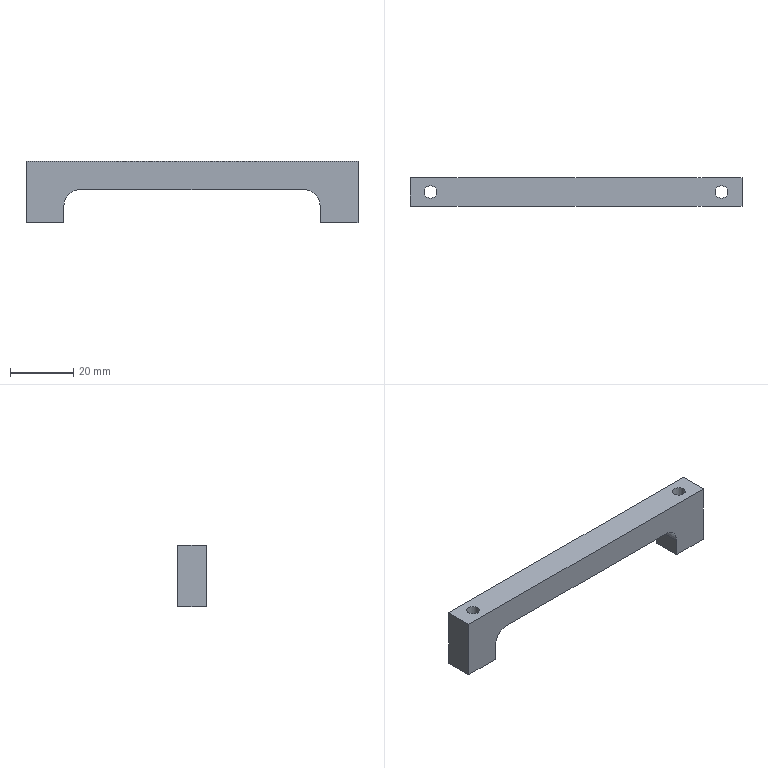Component | NX | LEG_2 | 1 solid | 14 faces | box 105 x 9 x 19.5 mm | volume 10379 mm3 | plane 10 | cylinder 4 | commonest cylinder face diameters 10 x2 4 x2
STEP:
#1=CARTESIAN_POINT('',(0.,0.,0.));
#2=DIRECTION('',(0.,0.,1.));
#3=DIRECTION('',(1.,0.,0.));
#4=AXIS2_PLACEMENT_3D('',#1,#2,#3);
#5=CARTESIAN_POINT('',(234.5,-71.5,106.5));
#6=VERTEX_POINT('',#5);
#7=CARTESIAN_POINT('',(230.5,-71.5,106.5));
#8=VERTEX_POINT('',#7);
#9=CARTESIAN_POINT('',(232.5,-71.5,106.5));
#10=DIRECTION('',(-0.,0.,-1.));
#11=DIRECTION('',(1.,0.,-0.));
#12=AXIS2_PLACEMENT_3D('',#9,#10,#11);
#13=CIRCLE('',#12,2.);
#14=CARTESIAN_POINT('',(278.5,-76.,106.5));
#15=DIRECTION('',(-0.,0.,-1.));
#16=DIRECTION('',(1.,0.,-0.));
#17=AXIS2_PLACEMENT_3D('',#14,#15,#16);
#18=PLANE('',#17);
#19=CARTESIAN_POINT('',(-46.,-4.5));
#20=DIRECTION('',(1.,0.));
#21=AXIS2_PLACEMENT_2D('',#19,#20);
#22=CIRCLE('',#21,2.);
#23=(GEOMETRIC_REPRESENTATION_CONTEXT(2)PARAMETRIC_REPRESENTATION_CONTEXT()REPRESENTATION_CONTEXT('',''));
#24=DEFINITIONAL_REPRESENTATION('',(#22),#23);
#25=PCURVE('',#18,#24);
#26=CARTESIAN_POINT('',(232.5,-71.5,86.5));
#27=DIRECTION('',(0.,0.,1.));
#28=DIRECTION('',(-1.,0.,0.));
#29=AXIS2_PLACEMENT_3D('',#26,#27,#28);
#30=CYLINDRICAL_SURFACE('',#29,2.);
#31=CARTESIAN_POINT('',(3.142,20.));
#32=DIRECTION('',(-1.,0.));
#33=VECTOR('',#32,1.);
#34=LINE('',#31,#33);
#35=(GEOMETRIC_REPRESENTATION_CONTEXT(2)PARAMETRIC_REPRESENTATION_CONTEXT()REPRESENTATION_CONTEXT('',''));
#36=DEFINITIONAL_REPRESENTATION('',(#34),#35);
#37=PCURVE('',#30,#36);
#38=SURFACE_CURVE('',#13,(#25,#37),.PCURVE_S1.);
#39=EDGE_CURVE('',#6,#8,#38,.T.);
#40=ORIENTED_EDGE('',*,*,#39,.T.);
#41=CARTESIAN_POINT('',(232.5,-71.5,106.5));
#42=DIRECTION('',(-0.,0.,-1.));
#43=DIRECTION('',(1.,0.,-0.));
#44=AXIS2_PLACEMENT_3D('',#41,#42,#43);
#45=CIRCLE('',#44,2.);
#46=CARTESIAN_POINT('',(-46.,-4.5));
#47=DIRECTION('',(1.,0.));
#48=AXIS2_PLACEMENT_2D('',#46,#47);
#49=CIRCLE('',#48,2.);
#50=(GEOMETRIC_REPRESENTATION_CONTEXT(2)PARAMETRIC_REPRESENTATION_CONTEXT()REPRESENTATION_CONTEXT('',''));
#51=DEFINITIONAL_REPRESENTATION('',(#49),#50);
#52=PCURVE('',#18,#51);
#53=CARTESIAN_POINT('',(9.425,20.));
#54=DIRECTION('',(-1.,0.));
#55=VECTOR('',#54,1.);
#56=LINE('',#53,#55);
#57=(GEOMETRIC_REPRESENTATION_CONTEXT(2)PARAMETRIC_REPRESENTATION_CONTEXT()REPRESENTATION_CONTEXT('',''));
#58=DEFINITIONAL_REPRESENTATION('',(#56),#57);
#59=PCURVE('',#30,#58);
#60=SURFACE_CURVE('',#45,(#52,#59),.PCURVE_S1.);
#61=EDGE_CURVE('',#8,#6,#60,.T.);
#62=ORIENTED_EDGE('',*,*,#61,.T.);
#63=EDGE_LOOP('',(#40,#62));
#64=FACE_BOUND('',#63,.T.);
#65=CARTESIAN_POINT('',(331.,-67.,106.5));
#66=VERTEX_POINT('',#65);
#67=CARTESIAN_POINT('',(226.,-67.,106.5));
#68=VERTEX_POINT('',#67);
#69=CARTESIAN_POINT('',(278.5,-67.,106.5));
#70=DIRECTION('',(-1.,0.,0.));
#71=VECTOR('',#70,1.);
#72=LINE('',#69,#71);
#73=CARTESIAN_POINT('',(0.,-9.));
#74=DIRECTION('',(-1.,0.));
#75=VECTOR('',#74,1.);
#76=LINE('',#73,#75);
#77=(GEOMETRIC_REPRESENTATION_CONTEXT(2)PARAMETRIC_REPRESENTATION_CONTEXT()REPRESENTATION_CONTEXT('',''));
#78=DEFINITIONAL_REPRESENTATION('',(#76),#77);
#79=PCURVE('',#18,#78);
#80=CARTESIAN_POINT('',(278.5,-67.,97.5));
#81=DIRECTION('',(0.,-1.,0.));
#82=DIRECTION('',(0.,0.,-1.));
#83=AXIS2_PLACEMENT_3D('',#80,#81,#82);
#84=PLANE('',#83);
#85=CARTESIAN_POINT('',(-9.,0.));
#86=DIRECTION('',(-0.,-1.));
#87=VECTOR('',#86,1.);
#88=LINE('',#85,#87);
#89=(GEOMETRIC_REPRESENTATION_CONTEXT(2)PARAMETRIC_REPRESENTATION_CONTEXT()REPRESENTATION_CONTEXT('',''));
#90=DEFINITIONAL_REPRESENTATION('',(#88),#89);
#91=PCURVE('',#84,#90);
#92=SURFACE_CURVE('',#72,(#79,#91),.PCURVE_S1.);
#93=EDGE_CURVE('',#66,#68,#92,.T.);
#94=ORIENTED_EDGE('',*,*,#93,.T.);
#95=CARTESIAN_POINT('',(226.,-76.,106.5));
#96=VERTEX_POINT('',#95);
#97=CARTESIAN_POINT('',(226.,-76.,106.5));
#98=DIRECTION('',(0.,1.,0.));
#99=VECTOR('',#98,1.);
#100=LINE('',#97,#99);
#101=CARTESIAN_POINT('',(-52.5,0.));
#102=DIRECTION('',(0.,-1.));
#103=VECTOR('',#102,1.);
#104=LINE('',#101,#103);
#105=(GEOMETRIC_REPRESENTATION_CONTEXT(2)PARAMETRIC_REPRESENTATION_CONTEXT()REPRESENTATION_CONTEXT('',''));
#106=DEFINITIONAL_REPRESENTATION('',(#104),#105);
#107=PCURVE('',#18,#106);
#108=CARTESIAN_POINT('',(226.,-76.,106.5));
#109=DIRECTION('',(1.,0.,0.));
#110=DIRECTION('',(0.,0.,1.));
#111=AXIS2_PLACEMENT_3D('',#108,#109,#110);
#112=PLANE('',#111);
#113=CARTESIAN_POINT('',(0.,0.));
#114=DIRECTION('',(0.,-1.));
#115=VECTOR('',#114,1.);
#116=LINE('',#113,#115);
#117=(GEOMETRIC_REPRESENTATION_CONTEXT(2)PARAMETRIC_REPRESENTATION_CONTEXT()REPRESENTATION_CONTEXT('',''));
#118=DEFINITIONAL_REPRESENTATION('',(#116),#117);
#119=PCURVE('',#112,#118);
#120=SURFACE_CURVE('',#100,(#107,#119),.PCURVE_S1.);
#121=EDGE_CURVE('',#96,#68,#120,.T.);
#122=ORIENTED_EDGE('',*,*,#121,.F.);
#123=CARTESIAN_POINT('',(331.,-76.,106.5));
#124=VERTEX_POINT('',#123);
#125=CARTESIAN_POINT('',(331.,-76.,106.5));
#126=DIRECTION('',(-1.,0.,-0.));
#127=VECTOR('',#126,1.);
#128=LINE('',#125,#127);
#129=CARTESIAN_POINT('',(52.5,0.));
#130=DIRECTION('',(-1.,0.));
#131=VECTOR('',#130,1.);
#132=LINE('',#129,#131);
#133=(GEOMETRIC_REPRESENTATION_CONTEXT(2)PARAMETRIC_REPRESENTATION_CONTEXT()REPRESENTATION_CONTEXT('',''));
#134=DEFINITIONAL_REPRESENTATION('',(#132),#133);
#135=PCURVE('',#18,#134);
#136=CARTESIAN_POINT('',(278.5,-76.,97.5));
#137=DIRECTION('',(0.,-1.,0.));
#138=DIRECTION('',(0.,0.,-1.));
#139=AXIS2_PLACEMENT_3D('',#136,#137,#138);
#140=PLANE('',#139);
#141=CARTESIAN_POINT('',(-9.,52.5));
#142=DIRECTION('',(0.,-1.));
#143=VECTOR('',#142,1.);
#144=LINE('',#141,#143);
#145=(GEOMETRIC_REPRESENTATION_CONTEXT(2)PARAMETRIC_REPRESENTATION_CONTEXT()REPRESENTATION_CONTEXT('',''));
#146=DEFINITIONAL_REPRESENTATION('',(#144),#145);
#147=PCURVE('',#140,#146);
#148=SURFACE_CURVE('',#128,(#135,#147),.PCURVE_S1.);
#149=EDGE_CURVE('',#124,#96,#148,.T.);
#150=ORIENTED_EDGE('',*,*,#149,.F.);
#151=CARTESIAN_POINT('',(331.,-76.,106.5));
#152=DIRECTION('',(0.,1.,0.));
#153=VECTOR('',#152,1.);
#154=LINE('',#151,#153);
#155=CARTESIAN_POINT('',(52.5,0.));
#156=DIRECTION('',(0.,-1.));
#157=VECTOR('',#156,1.);
#158=LINE('',#155,#157);
#159=(GEOMETRIC_REPRESENTATION_CONTEXT(2)PARAMETRIC_REPRESENTATION_CONTEXT()REPRESENTATION_CONTEXT('',''));
#160=DEFINITIONAL_REPRESENTATION('',(#158),#159);
#161=PCURVE('',#18,#160);
#162=CARTESIAN_POINT('',(331.,-76.,87.));
#163=DIRECTION('',(-1.,0.,0.));
#164=DIRECTION('',(0.,0.,-1.));
#165=AXIS2_PLACEMENT_3D('',#162,#163,#164);
#166=PLANE('',#165);
#167=CARTESIAN_POINT('',(-19.5,0.));
#168=DIRECTION('',(0.,-1.));
#169=VECTOR('',#168,1.);
#170=LINE('',#167,#169);
#171=(GEOMETRIC_REPRESENTATION_CONTEXT(2)PARAMETRIC_REPRESENTATION_CONTEXT()REPRESENTATION_CONTEXT('',''));
#172=DEFINITIONAL_REPRESENTATION('',(#170),#171);
#173=PCURVE('',#166,#172);
#174=SURFACE_CURVE('',#154,(#161,#173),.PCURVE_S1.);
#175=EDGE_CURVE('',#124,#66,#174,.T.);
#176=ORIENTED_EDGE('',*,*,#175,.T.);
#177=EDGE_LOOP('',(#94,#122,#150,#176));
#178=FACE_BOUND('',#177,.T.);
#179=CARTESIAN_POINT('',(322.5,-71.5,106.5));
#180=VERTEX_POINT('',#179);
#181=CARTESIAN_POINT('',(324.5,-71.5,106.5));
#182=DIRECTION('',(0.,0.,1.));
#183=DIRECTION('',(-1.,0.,0.));
#184=AXIS2_PLACEMENT_3D('',#181,#182,#183);
#185=CIRCLE('',#184,2.);
#186=CARTESIAN_POINT('',(44.,-4.5));
#187=CARTESIAN_POINT('',(44.,-1.036));
#188=CARTESIAN_POINT('',(47.,-2.768));
#189=CARTESIAN_POINT('',(50.,-4.5));
#190=CARTESIAN_POINT('',(47.,-6.232));
#191=CARTESIAN_POINT('',(44.,-7.964));
#192=CARTESIAN_POINT('',(44.,-4.5));
#193=(BOUNDED_CURVE()B_SPLINE_CURVE(2,(#186,#187,#188,#189,#190,#191,#192),.UNSPECIFIED.,.T.,.F.)B_SPLINE_CURVE_WITH_KNOTS((1,2,2,2,2,1),(-2.094,0.,2.094,4.189,6.283,8.378),.UNSPECIFIED.)CURVE()GEOMETRIC_REPRESENTATION_ITEM()RATIONAL_B_SPLINE_CURVE((1.,0.5,1.,0.5,1.,0.5,1.))REPRESENTATION_ITEM(''));
#194=(GEOMETRIC_REPRESENTATION_CONTEXT(2)PARAMETRIC_REPRESENTATION_CONTEXT()REPRESENTATION_CONTEXT('',''));
#195=DEFINITIONAL_REPRESENTATION('',(#193),#194);
#196=PCURVE('',#18,#195);
#197=CARTESIAN_POINT('',(324.5,-71.5,86.5));
#198=DIRECTION('',(0.,0.,1.));
#199=DIRECTION('',(-1.,0.,0.));
#200=AXIS2_PLACEMENT_3D('',#197,#198,#199);
#201=CYLINDRICAL_SURFACE('',#200,2.);
#202=CARTESIAN_POINT('',(0.,20.));
#203=DIRECTION('',(1.,0.));
#204=VECTOR('',#203,1.);
#205=LINE('',#202,#204);
#206=(GEOMETRIC_REPRESENTATION_CONTEXT(2)PARAMETRIC_REPRESENTATION_CONTEXT()REPRESENTATION_CONTEXT('',''));
#207=DEFINITIONAL_REPRESENTATION('',(#205),#206);
#208=PCURVE('',#201,#207);
#209=SURFACE_CURVE('',#185,(#196,#208),.PCURVE_S1.);
#210=EDGE_CURVE('',#180,#180,#209,.T.);
#211=ORIENTED_EDGE('',*,*,#210,.F.);
#212=EDGE_LOOP('',(#211));
#213=FACE_BOUND('',#212,.T.);
#214=ADVANCED_FACE('',(#64,#178,#213),#18,.F.);
#215=CARTESIAN_POINT('',(331.,-67.,87.));
#216=VERTEX_POINT('',#215);
#217=CARTESIAN_POINT('',(331.,-67.,87.));
#218=DIRECTION('',(0.,0.,1.));
#219=VECTOR('',#218,1.);
#220=LINE('',#217,#219);
#221=CARTESIAN_POINT('',(0.,-9.));
#222=DIRECTION('',(-1.,0.));
#223=VECTOR('',#222,1.);
#224=LINE('',#221,#223);
#225=(GEOMETRIC_REPRESENTATION_CONTEXT(2)PARAMETRIC_REPRESENTATION_CONTEXT()REPRESENTATION_CONTEXT('',''));
#226=DEFINITIONAL_REPRESENTATION('',(#224),#225);
#227=PCURVE('',#166,#226);
#228=CARTESIAN_POINT('',(10.5,52.5));
#229=DIRECTION('',(-1.,0.));
#230=VECTOR('',#229,1.);
#231=LINE('',#228,#230);
#232=(GEOMETRIC_REPRESENTATION_CONTEXT(2)PARAMETRIC_REPRESENTATION_CONTEXT()REPRESENTATION_CONTEXT('',''));
#233=DEFINITIONAL_REPRESENTATION('',(#231),#232);
#234=PCURVE('',#84,#233);
#235=SURFACE_CURVE('',#220,(#227,#234),.PCURVE_S1.);
#236=EDGE_CURVE('',#216,#66,#235,.T.);
#237=ORIENTED_EDGE('',*,*,#236,.T.);
#238=ORIENTED_EDGE('',*,*,#175,.F.);
#239=CARTESIAN_POINT('',(331.,-76.,87.));
#240=VERTEX_POINT('',#239);
#241=CARTESIAN_POINT('',(331.,-76.,87.));
#242=DIRECTION('',(0.,0.,1.));
#243=VECTOR('',#242,1.);
#244=LINE('',#241,#243);
#245=CARTESIAN_POINT('',(0.,0.));
#246=DIRECTION('',(-1.,0.));
#247=VECTOR('',#246,1.);
#248=LINE('',#245,#247);
#249=(GEOMETRIC_REPRESENTATION_CONTEXT(2)PARAMETRIC_REPRESENTATION_CONTEXT()REPRESENTATION_CONTEXT('',''));
#250=DEFINITIONAL_REPRESENTATION('',(#248),#249);
#251=PCURVE('',#166,#250);
#252=CARTESIAN_POINT('',(10.5,52.5));
#253=DIRECTION('',(-1.,0.));
#254=VECTOR('',#253,1.);
#255=LINE('',#252,#254);
#256=(GEOMETRIC_REPRESENTATION_CONTEXT(2)PARAMETRIC_REPRESENTATION_CONTEXT()REPRESENTATION_CONTEXT('',''));
#257=DEFINITIONAL_REPRESENTATION('',(#255),#256);
#258=PCURVE('',#140,#257);
#259=SURFACE_CURVE('',#244,(#251,#258),.PCURVE_S1.);
#260=EDGE_CURVE('',#240,#124,#259,.T.);
#261=ORIENTED_EDGE('',*,*,#260,.F.);
#262=CARTESIAN_POINT('',(331.,-76.,87.));
#263=DIRECTION('',(0.,1.,0.));
#264=VECTOR('',#263,1.);
#265=LINE('',#262,#264);
#266=CARTESIAN_POINT('',(0.,0.));
#267=DIRECTION('',(0.,-1.));
#268=VECTOR('',#267,1.);
#269=LINE('',#266,#268);
#270=(GEOMETRIC_REPRESENTATION_CONTEXT(2)PARAMETRIC_REPRESENTATION_CONTEXT()REPRESENTATION_CONTEXT('',''));
#271=DEFINITIONAL_REPRESENTATION('',(#269),#270);
#272=PCURVE('',#166,#271);
#273=CARTESIAN_POINT('',(319.,-76.,87.));
#274=DIRECTION('',(0.,0.,1.));
#275=DIRECTION('',(-1.,0.,0.));
#276=AXIS2_PLACEMENT_3D('',#273,#274,#275);
#277=PLANE('',#276);
#278=CARTESIAN_POINT('',(-12.,0.));
#279=DIRECTION('',(0.,-1.));
#280=VECTOR('',#279,1.);
#281=LINE('',#278,#280);
#282=(GEOMETRIC_REPRESENTATION_CONTEXT(2)PARAMETRIC_REPRESENTATION_CONTEXT()REPRESENTATION_CONTEXT('',''));
#283=DEFINITIONAL_REPRESENTATION('',(#281),#282);
#284=PCURVE('',#277,#283);
#285=SURFACE_CURVE('',#265,(#272,#284),.PCURVE_S1.);
#286=EDGE_CURVE('',#240,#216,#285,.T.);
#287=ORIENTED_EDGE('',*,*,#286,.T.);
#288=EDGE_LOOP('',(#237,#238,#261,#287));
#289=FACE_BOUND('',#288,.T.);
#290=ADVANCED_FACE('',(#289),#166,.F.);
#291=CARTESIAN_POINT('',(226.,-67.,87.));
#292=VERTEX_POINT('',#291);
#293=CARTESIAN_POINT('',(226.,-67.,106.5));
#294=DIRECTION('',(0.,0.,-1.));
#295=VECTOR('',#294,1.);
#296=LINE('',#293,#295);
#297=CARTESIAN_POINT('',(0.,-9.));
#298=DIRECTION('',(-1.,0.));
#299=VECTOR('',#298,1.);
#300=LINE('',#297,#299);
#301=(GEOMETRIC_REPRESENTATION_CONTEXT(2)PARAMETRIC_REPRESENTATION_CONTEXT()REPRESENTATION_CONTEXT('',''));
#302=DEFINITIONAL_REPRESENTATION('',(#300),#301);
#303=PCURVE('',#112,#302);
#304=CARTESIAN_POINT('',(-9.,-52.5));
#305=DIRECTION('',(1.,0.));
#306=VECTOR('',#305,1.);
#307=LINE('',#304,#306);
#308=(GEOMETRIC_REPRESENTATION_CONTEXT(2)PARAMETRIC_REPRESENTATION_CONTEXT()REPRESENTATION_CONTEXT('',''));
#309=DEFINITIONAL_REPRESENTATION('',(#307),#308);
#310=PCURVE('',#84,#309);
#311=SURFACE_CURVE('',#296,(#303,#310),.PCURVE_S1.);
#312=EDGE_CURVE('',#68,#292,#311,.T.);
#313=ORIENTED_EDGE('',*,*,#312,.T.);
#314=CARTESIAN_POINT('',(226.,-76.,87.));
#315=VERTEX_POINT('',#314);
#316=CARTESIAN_POINT('',(226.,-76.,87.));
#317=DIRECTION('',(0.,1.,0.));
#318=VECTOR('',#317,1.);
#319=LINE('',#316,#318);
#320=CARTESIAN_POINT('',(-19.5,0.));
#321=DIRECTION('',(0.,-1.));
#322=VECTOR('',#321,1.);
#323=LINE('',#320,#322);
#324=(GEOMETRIC_REPRESENTATION_CONTEXT(2)PARAMETRIC_REPRESENTATION_CONTEXT()REPRESENTATION_CONTEXT('',''));
#325=DEFINITIONAL_REPRESENTATION('',(#323),#324);
#326=PCURVE('',#112,#325);
#327=CARTESIAN_POINT('',(226.,-76.,87.));
#328=DIRECTION('',(-0.,0.,1.));
#329=DIRECTION('',(-1.,0.,-0.));
#330=AXIS2_PLACEMENT_3D('',#327,#328,#329);
#331=PLANE('',#330);
#332=CARTESIAN_POINT('',(0.,0.));
#333=DIRECTION('',(0.,-1.));
#334=VECTOR('',#333,1.);
#335=LINE('',#332,#334);
#336=(GEOMETRIC_REPRESENTATION_CONTEXT(2)PARAMETRIC_REPRESENTATION_CONTEXT()REPRESENTATION_CONTEXT('',''));
#337=DEFINITIONAL_REPRESENTATION('',(#335),#336);
#338=PCURVE('',#331,#337);
#339=SURFACE_CURVE('',#319,(#326,#338),.PCURVE_S1.);
#340=EDGE_CURVE('',#315,#292,#339,.T.);
#341=ORIENTED_EDGE('',*,*,#340,.F.);
#342=CARTESIAN_POINT('',(226.,-76.,106.5));
#343=DIRECTION('',(0.,0.,-1.));
#344=VECTOR('',#343,1.);
#345=LINE('',#342,#344);
#346=CARTESIAN_POINT('',(0.,0.));
#347=DIRECTION('',(-1.,0.));
#348=VECTOR('',#347,1.);
#349=LINE('',#346,#348);
#350=(GEOMETRIC_REPRESENTATION_CONTEXT(2)PARAMETRIC_REPRESENTATION_CONTEXT()REPRESENTATION_CONTEXT('',''));
#351=DEFINITIONAL_REPRESENTATION('',(#349),#350);
#352=PCURVE('',#112,#351);
#353=CARTESIAN_POINT('',(-9.,-52.5));
#354=DIRECTION('',(1.,0.));
#355=VECTOR('',#354,1.);
#356=LINE('',#353,#355);
#357=(GEOMETRIC_REPRESENTATION_CONTEXT(2)PARAMETRIC_REPRESENTATION_CONTEXT()REPRESENTATION_CONTEXT('',''));
#358=DEFINITIONAL_REPRESENTATION('',(#356),#357);
#359=PCURVE('',#140,#358);
#360=SURFACE_CURVE('',#345,(#352,#359),.PCURVE_S1.);
#361=EDGE_CURVE('',#96,#315,#360,.T.);
#362=ORIENTED_EDGE('',*,*,#361,.F.);
#363=ORIENTED_EDGE('',*,*,#121,.T.);
#364=EDGE_LOOP('',(#313,#341,#362,#363));
#365=FACE_BOUND('',#364,.T.);
#366=ADVANCED_FACE('',(#365),#112,.F.);
#367=CARTESIAN_POINT('',(230.5,-71.5,87.));
#368=VERTEX_POINT('',#367);
#369=CARTESIAN_POINT('',(232.5,-71.5,87.));
#370=DIRECTION('',(0.,0.,-1.));
#371=DIRECTION('',(-1.,0.,-0.));
#372=AXIS2_PLACEMENT_3D('',#369,#370,#371);
#373=CIRCLE('',#372,2.);
#374=CARTESIAN_POINT('',(-4.5,-4.5));
#375=CARTESIAN_POINT('',(-4.5,-7.964));
#376=CARTESIAN_POINT('',(-7.5,-6.232));
#377=CARTESIAN_POINT('',(-10.5,-4.5));
#378=CARTESIAN_POINT('',(-7.5,-2.768));
#379=CARTESIAN_POINT('',(-4.5,-1.036));
#380=CARTESIAN_POINT('',(-4.5,-4.5));
#381=(BOUNDED_CURVE()B_SPLINE_CURVE(2,(#374,#375,#376,#377,#378,#379,#380),.UNSPECIFIED.,.T.,.F.)B_SPLINE_CURVE_WITH_KNOTS((1,2,2,2,2,1),(-2.094,0.,2.094,4.189,6.283,8.378),.UNSPECIFIED.)CURVE()GEOMETRIC_REPRESENTATION_ITEM()RATIONAL_B_SPLINE_CURVE((1.,0.5,1.,0.5,1.,0.5,1.))REPRESENTATION_ITEM(''));
#382=(GEOMETRIC_REPRESENTATION_CONTEXT(2)PARAMETRIC_REPRESENTATION_CONTEXT()REPRESENTATION_CONTEXT('',''));
#383=DEFINITIONAL_REPRESENTATION('',(#381),#382);
#384=PCURVE('',#331,#383);
#385=CARTESIAN_POINT('',(6.283,0.5));
#386=DIRECTION('',(-1.,0.));
#387=VECTOR('',#386,1.);
#388=LINE('',#385,#387);
#389=(GEOMETRIC_REPRESENTATION_CONTEXT(2)PARAMETRIC_REPRESENTATION_CONTEXT()REPRESENTATION_CONTEXT('',''));
#390=DEFINITIONAL_REPRESENTATION('',(#388),#389);
#391=PCURVE('',#30,#390);
#392=SURFACE_CURVE('',#373,(#384,#391),.PCURVE_S1.);
#393=EDGE_CURVE('',#368,#368,#392,.T.);
#394=ORIENTED_EDGE('',*,*,#393,.F.);
#395=EDGE_LOOP('',(#394));
#396=FACE_BOUND('',#395,.T.);
#397=CARTESIAN_POINT('',(238.,-67.,87.));
#398=VERTEX_POINT('',#397);
#399=CARTESIAN_POINT('',(226.,-67.,87.));
#400=DIRECTION('',(1.,0.,0.));
#401=VECTOR('',#400,1.);
#402=LINE('',#399,#401);
#403=CARTESIAN_POINT('',(0.,-9.));
#404=DIRECTION('',(-1.,0.));
#405=VECTOR('',#404,1.);
#406=LINE('',#403,#405);
#407=(GEOMETRIC_REPRESENTATION_CONTEXT(2)PARAMETRIC_REPRESENTATION_CONTEXT()REPRESENTATION_CONTEXT('',''));
#408=DEFINITIONAL_REPRESENTATION('',(#406),#407);
#409=PCURVE('',#331,#408);
#410=CARTESIAN_POINT('',(10.5,-52.5));
#411=DIRECTION('',(-0.,1.));
#412=VECTOR('',#411,1.);
#413=LINE('',#410,#412);
#414=(GEOMETRIC_REPRESENTATION_CONTEXT(2)PARAMETRIC_REPRESENTATION_CONTEXT()REPRESENTATION_CONTEXT('',''));
#415=DEFINITIONAL_REPRESENTATION('',(#413),#414);
#416=PCURVE('',#84,#415);
#417=SURFACE_CURVE('',#402,(#409,#416),.PCURVE_S1.);
#418=EDGE_CURVE('',#292,#398,#417,.T.);
#419=ORIENTED_EDGE('',*,*,#418,.T.);
#420=CARTESIAN_POINT('',(238.,-76.,87.));
#421=VERTEX_POINT('',#420);
#422=CARTESIAN_POINT('',(238.,-76.,87.));
#423=DIRECTION('',(0.,1.,0.));
#424=VECTOR('',#423,1.);
#425=LINE('',#422,#424);
#426=CARTESIAN_POINT('',(-12.,0.));
#427=DIRECTION('',(0.,-1.));
#428=VECTOR('',#427,1.);
#429=LINE('',#426,#428);
#430=(GEOMETRIC_REPRESENTATION_CONTEXT(2)PARAMETRIC_REPRESENTATION_CONTEXT()REPRESENTATION_CONTEXT('',''));
#431=DEFINITIONAL_REPRESENTATION('',(#429),#430);
#432=PCURVE('',#331,#431);
#433=CARTESIAN_POINT('',(238.,-76.,87.));
#434=DIRECTION('',(-1.,0.,0.));
#435=DIRECTION('',(0.,0.,-1.));
#436=AXIS2_PLACEMENT_3D('',#433,#434,#435);
#437=PLANE('',#436);
#438=CARTESIAN_POINT('',(0.,0.));
#439=DIRECTION('',(0.,-1.));
#440=VECTOR('',#439,1.);
#441=LINE('',#438,#440);
#442=(GEOMETRIC_REPRESENTATION_CONTEXT(2)PARAMETRIC_REPRESENTATION_CONTEXT()REPRESENTATION_CONTEXT('',''));
#443=DEFINITIONAL_REPRESENTATION('',(#441),#442);
#444=PCURVE('',#437,#443);
#445=SURFACE_CURVE('',#425,(#432,#444),.PCURVE_S1.);
#446=EDGE_CURVE('',#421,#398,#445,.T.);
#447=ORIENTED_EDGE('',*,*,#446,.F.);
#448=CARTESIAN_POINT('',(226.,-76.,87.));
#449=DIRECTION('',(1.,0.,0.));
#450=VECTOR('',#449,1.);
#451=LINE('',#448,#450);
#452=CARTESIAN_POINT('',(0.,0.));
#453=DIRECTION('',(-1.,0.));
#454=VECTOR('',#453,1.);
#455=LINE('',#452,#454);
#456=(GEOMETRIC_REPRESENTATION_CONTEXT(2)PARAMETRIC_REPRESENTATION_CONTEXT()REPRESENTATION_CONTEXT('',''));
#457=DEFINITIONAL_REPRESENTATION('',(#455),#456);
#458=PCURVE('',#331,#457);
#459=CARTESIAN_POINT('',(10.5,-52.5));
#460=DIRECTION('',(-0.,1.));
#461=VECTOR('',#460,1.);
#462=LINE('',#459,#461);
#463=(GEOMETRIC_REPRESENTATION_CONTEXT(2)PARAMETRIC_REPRESENTATION_CONTEXT()REPRESENTATION_CONTEXT('',''));
#464=DEFINITIONAL_REPRESENTATION('',(#462),#463);
#465=PCURVE('',#140,#464);
#466=SURFACE_CURVE('',#451,(#458,#465),.PCURVE_S1.);
#467=EDGE_CURVE('',#315,#421,#466,.T.);
#468=ORIENTED_EDGE('',*,*,#467,.F.);
#469=ORIENTED_EDGE('',*,*,#340,.T.);
#470=EDGE_LOOP('',(#419,#447,#468,#469));
#471=FACE_BOUND('',#470,.T.);
#472=ADVANCED_FACE('',(#396,#471),#331,.F.);
#473=CARTESIAN_POINT('',(238.,-67.,92.5));
#474=VERTEX_POINT('',#473);
#475=CARTESIAN_POINT('',(238.,-67.,87.));
#476=DIRECTION('',(0.,0.,1.));
#477=VECTOR('',#476,1.);
#478=LINE('',#475,#477);
#479=CARTESIAN_POINT('',(0.,-9.));
#480=DIRECTION('',(-1.,0.));
#481=VECTOR('',#480,1.);
#482=LINE('',#479,#481);
#483=(GEOMETRIC_REPRESENTATION_CONTEXT(2)PARAMETRIC_REPRESENTATION_CONTEXT()REPRESENTATION_CONTEXT('',''));
#484=DEFINITIONAL_REPRESENTATION('',(#482),#483);
#485=PCURVE('',#437,#484);
#486=CARTESIAN_POINT('',(10.5,-40.5));
#487=DIRECTION('',(-1.,0.));
#488=VECTOR('',#487,1.);
#489=LINE('',#486,#488);
#490=(GEOMETRIC_REPRESENTATION_CONTEXT(2)PARAMETRIC_REPRESENTATION_CONTEXT()REPRESENTATION_CONTEXT('',''));
#491=DEFINITIONAL_REPRESENTATION('',(#489),#490);
#492=PCURVE('',#84,#491);
#493=SURFACE_CURVE('',#478,(#485,#492),.PCURVE_S1.);
#494=EDGE_CURVE('',#398,#474,#493,.T.);
#495=ORIENTED_EDGE('',*,*,#494,.T.);
#496=CARTESIAN_POINT('',(238.,-76.,92.5));
#497=VERTEX_POINT('',#496);
#498=CARTESIAN_POINT('',(238.,-76.,92.5));
#499=DIRECTION('',(0.,-1.,0.));
#500=VECTOR('',#499,1.);
#501=LINE('',#498,#500);
#502=CARTESIAN_POINT('',(-5.5,0.));
#503=DIRECTION('',(0.,1.));
#504=VECTOR('',#503,1.);
#505=LINE('',#502,#504);
#506=(GEOMETRIC_REPRESENTATION_CONTEXT(2)PARAMETRIC_REPRESENTATION_CONTEXT()REPRESENTATION_CONTEXT('',''));
#507=DEFINITIONAL_REPRESENTATION('',(#505),#506);
#508=PCURVE('',#437,#507);
#509=CARTESIAN_POINT('',(243.,-76.,92.5));
#510=DIRECTION('',(0.,-1.,0.));
#511=DIRECTION('',(0.,0.,-1.));
#512=AXIS2_PLACEMENT_3D('',#509,#510,#511);
#513=CYLINDRICAL_SURFACE('',#512,5.);
#514=CARTESIAN_POINT('',(4.712,0.));
#515=DIRECTION('',(0.,1.));
#516=VECTOR('',#515,1.);
#517=LINE('',#514,#516);
#518=(GEOMETRIC_REPRESENTATION_CONTEXT(2)PARAMETRIC_REPRESENTATION_CONTEXT()REPRESENTATION_CONTEXT('',''));
#519=DEFINITIONAL_REPRESENTATION('',(#517),#518);
#520=PCURVE('',#513,#519);
#521=SURFACE_CURVE('',#501,(#508,#520),.PCURVE_S1.);
#522=EDGE_CURVE('',#474,#497,#521,.T.);
#523=ORIENTED_EDGE('',*,*,#522,.T.);
#524=CARTESIAN_POINT('',(238.,-76.,87.));
#525=DIRECTION('',(0.,0.,1.));
#526=VECTOR('',#525,1.);
#527=LINE('',#524,#526);
#528=CARTESIAN_POINT('',(0.,0.));
#529=DIRECTION('',(-1.,0.));
#530=VECTOR('',#529,1.);
#531=LINE('',#528,#530);
#532=(GEOMETRIC_REPRESENTATION_CONTEXT(2)PARAMETRIC_REPRESENTATION_CONTEXT()REPRESENTATION_CONTEXT('',''));
#533=DEFINITIONAL_REPRESENTATION('',(#531),#532);
#534=PCURVE('',#437,#533);
#535=CARTESIAN_POINT('',(10.5,-40.5));
#536=DIRECTION('',(-1.,0.));
#537=VECTOR('',#536,1.);
#538=LINE('',#535,#537);
#539=(GEOMETRIC_REPRESENTATION_CONTEXT(2)PARAMETRIC_REPRESENTATION_CONTEXT()REPRESENTATION_CONTEXT('',''));
#540=DEFINITIONAL_REPRESENTATION('',(#538),#539);
#541=PCURVE('',#140,#540);
#542=SURFACE_CURVE('',#527,(#534,#541),.PCURVE_S1.);
#543=EDGE_CURVE('',#421,#497,#542,.T.);
#544=ORIENTED_EDGE('',*,*,#543,.F.);
#545=ORIENTED_EDGE('',*,*,#446,.T.);
#546=EDGE_LOOP('',(#495,#523,#544,#545));
#547=FACE_BOUND('',#546,.T.);
#548=ADVANCED_FACE('',(#547),#437,.F.);
#549=CARTESIAN_POINT('',(243.,-67.,97.5));
#550=VERTEX_POINT('',#549);
#551=CARTESIAN_POINT('',(314.,-67.,97.5));
#552=VERTEX_POINT('',#551);
#553=CARTESIAN_POINT('',(278.5,-67.,97.5));
#554=DIRECTION('',(1.,0.,-0.));
#555=VECTOR('',#554,1.);
#556=LINE('',#553,#555);
#557=CARTESIAN_POINT('',(278.5,-76.,97.5));
#558=DIRECTION('',(0.,0.,1.));
#559=DIRECTION('',(-1.,0.,0.));
#560=AXIS2_PLACEMENT_3D('',#557,#558,#559);
#561=PLANE('',#560);
#562=CARTESIAN_POINT('',(0.,-9.));
#563=DIRECTION('',(-1.,0.));
#564=VECTOR('',#563,1.);
#565=LINE('',#562,#564);
#566=(GEOMETRIC_REPRESENTATION_CONTEXT(2)PARAMETRIC_REPRESENTATION_CONTEXT()REPRESENTATION_CONTEXT('',''));
#567=DEFINITIONAL_REPRESENTATION('',(#565),#566);
#568=PCURVE('',#561,#567);
#569=CARTESIAN_POINT('',(0.,0.));
#570=DIRECTION('',(0.,1.));
#571=VECTOR('',#570,1.);
#572=LINE('',#569,#571);
#573=(GEOMETRIC_REPRESENTATION_CONTEXT(2)PARAMETRIC_REPRESENTATION_CONTEXT()REPRESENTATION_CONTEXT('',''));
#574=DEFINITIONAL_REPRESENTATION('',(#572),#573);
#575=PCURVE('',#84,#574);
#576=SURFACE_CURVE('',#556,(#568,#575),.PCURVE_S1.);
#577=EDGE_CURVE('',#550,#552,#576,.T.);
#578=ORIENTED_EDGE('',*,*,#577,.T.);
#579=CARTESIAN_POINT('',(314.,-76.,97.5));
#580=VERTEX_POINT('',#579);
#581=CARTESIAN_POINT('',(314.,-76.,97.5));
#582=DIRECTION('',(0.,-1.,0.));
#583=VECTOR('',#582,1.);
#584=LINE('',#581,#583);
#585=CARTESIAN_POINT('',(-35.5,0.));
#586=DIRECTION('',(0.,1.));
#587=VECTOR('',#586,1.);
#588=LINE('',#585,#587);
#589=(GEOMETRIC_REPRESENTATION_CONTEXT(2)PARAMETRIC_REPRESENTATION_CONTEXT()REPRESENTATION_CONTEXT('',''));
#590=DEFINITIONAL_REPRESENTATION('',(#588),#589);
#591=PCURVE('',#561,#590);
#592=CARTESIAN_POINT('',(314.,-76.,92.5));
#593=DIRECTION('',(0.,-1.,0.));
#594=DIRECTION('',(0.,0.,-1.));
#595=AXIS2_PLACEMENT_3D('',#592,#593,#594);
#596=CYLINDRICAL_SURFACE('',#595,5.);
#597=CARTESIAN_POINT('',(3.142,0.));
#598=DIRECTION('',(0.,1.));
#599=VECTOR('',#598,1.);
#600=LINE('',#597,#599);
#601=(GEOMETRIC_REPRESENTATION_CONTEXT(2)PARAMETRIC_REPRESENTATION_CONTEXT()REPRESENTATION_CONTEXT('',''));
#602=DEFINITIONAL_REPRESENTATION('',(#600),#601);
#603=PCURVE('',#596,#602);
#604=SURFACE_CURVE('',#584,(#591,#603),.PCURVE_S1.);
#605=EDGE_CURVE('',#552,#580,#604,.T.);
#606=ORIENTED_EDGE('',*,*,#605,.T.);
#607=CARTESIAN_POINT('',(243.,-76.,97.5));
#608=VERTEX_POINT('',#607);
#609=CARTESIAN_POINT('',(238.,-76.,97.5));
#610=DIRECTION('',(1.,0.,0.));
#611=VECTOR('',#610,1.);
#612=LINE('',#609,#611);
#613=CARTESIAN_POINT('',(40.5,0.));
#614=DIRECTION('',(-1.,0.));
#615=VECTOR('',#614,1.);
#616=LINE('',#613,#615);
#617=(GEOMETRIC_REPRESENTATION_CONTEXT(2)PARAMETRIC_REPRESENTATION_CONTEXT()REPRESENTATION_CONTEXT('',''));
#618=DEFINITIONAL_REPRESENTATION('',(#616),#617);
#619=PCURVE('',#561,#618);
#620=CARTESIAN_POINT('',(0.,-40.5));
#621=DIRECTION('',(-0.,1.));
#622=VECTOR('',#621,1.);
#623=LINE('',#620,#622);
#624=(GEOMETRIC_REPRESENTATION_CONTEXT(2)PARAMETRIC_REPRESENTATION_CONTEXT()REPRESENTATION_CONTEXT('',''));
#625=DEFINITIONAL_REPRESENTATION('',(#623),#624);
#626=PCURVE('',#140,#625);
#627=SURFACE_CURVE('',#612,(#619,#626),.PCURVE_S1.);
#628=EDGE_CURVE('',#608,#580,#627,.T.);
#629=ORIENTED_EDGE('',*,*,#628,.F.);
#630=CARTESIAN_POINT('',(243.,-67.,97.5));
#631=DIRECTION('',(0.,1.,0.));
#632=VECTOR('',#631,1.);
#633=LINE('',#630,#632);
#634=CARTESIAN_POINT('',(35.5,-9.));
#635=DIRECTION('',(0.,-1.));
#636=VECTOR('',#635,1.);
#637=LINE('',#634,#636);
#638=(GEOMETRIC_REPRESENTATION_CONTEXT(2)PARAMETRIC_REPRESENTATION_CONTEXT()REPRESENTATION_CONTEXT('',''));
#639=DEFINITIONAL_REPRESENTATION('',(#637),#638);
#640=PCURVE('',#561,#639);
#641=CARTESIAN_POINT('',(3.142,-9.));
#642=DIRECTION('',(0.,-1.));
#643=VECTOR('',#642,1.);
#644=LINE('',#641,#643);
#645=(GEOMETRIC_REPRESENTATION_CONTEXT(2)PARAMETRIC_REPRESENTATION_CONTEXT()REPRESENTATION_CONTEXT('',''));
#646=DEFINITIONAL_REPRESENTATION('',(#644),#645);
#647=PCURVE('',#513,#646);
#648=SURFACE_CURVE('',#633,(#640,#647),.PCURVE_S1.);
#649=EDGE_CURVE('',#608,#550,#648,.T.);
#650=ORIENTED_EDGE('',*,*,#649,.T.);
#651=EDGE_LOOP('',(#578,#606,#629,#650));
#652=FACE_BOUND('',#651,.T.);
#653=ADVANCED_FACE('',(#652),#561,.F.);
#654=CARTESIAN_POINT('',(319.,-76.,92.5));
#655=VERTEX_POINT('',#654);
#656=CARTESIAN_POINT('',(319.,-76.,87.));
#657=VERTEX_POINT('',#656);
#658=CARTESIAN_POINT('',(319.,-76.,97.5));
#659=DIRECTION('',(0.,0.,-1.));
#660=VECTOR('',#659,1.);
#661=LINE('',#658,#660);
#662=CARTESIAN_POINT('',(319.,-76.,97.5));
#663=DIRECTION('',(1.,0.,0.));
#664=DIRECTION('',(0.,0.,1.));
#665=AXIS2_PLACEMENT_3D('',#662,#663,#664);
#666=PLANE('',#665);
#667=CARTESIAN_POINT('',(0.,0.));
#668=DIRECTION('',(-1.,0.));
#669=VECTOR('',#668,1.);
#670=LINE('',#667,#669);
#671=(GEOMETRIC_REPRESENTATION_CONTEXT(2)PARAMETRIC_REPRESENTATION_CONTEXT()REPRESENTATION_CONTEXT('',''));
#672=DEFINITIONAL_REPRESENTATION('',(#670),#671);
#673=PCURVE('',#666,#672);
#674=CARTESIAN_POINT('',(0.,40.5));
#675=DIRECTION('',(1.,0.));
#676=VECTOR('',#675,1.);
#677=LINE('',#674,#676);
#678=(GEOMETRIC_REPRESENTATION_CONTEXT(2)PARAMETRIC_REPRESENTATION_CONTEXT()REPRESENTATION_CONTEXT('',''));
#679=DEFINITIONAL_REPRESENTATION('',(#677),#678);
#680=PCURVE('',#140,#679);
#681=SURFACE_CURVE('',#661,(#673,#680),.PCURVE_S1.);
#682=EDGE_CURVE('',#655,#657,#681,.T.);
#683=ORIENTED_EDGE('',*,*,#682,.F.);
#684=CARTESIAN_POINT('',(319.,-67.,92.5));
#685=VERTEX_POINT('',#684);
#686=CARTESIAN_POINT('',(319.,-67.,92.5));
#687=DIRECTION('',(0.,1.,0.));
#688=VECTOR('',#687,1.);
#689=LINE('',#686,#688);
#690=CARTESIAN_POINT('',(-5.,-9.));
#691=DIRECTION('',(0.,-1.));
#692=VECTOR('',#691,1.);
#693=LINE('',#690,#692);
#694=(GEOMETRIC_REPRESENTATION_CONTEXT(2)PARAMETRIC_REPRESENTATION_CONTEXT()REPRESENTATION_CONTEXT('',''));
#695=DEFINITIONAL_REPRESENTATION('',(#693),#694);
#696=PCURVE('',#666,#695);
#697=CARTESIAN_POINT('',(1.571,-9.));
#698=DIRECTION('',(0.,-1.));
#699=VECTOR('',#698,1.);
#700=LINE('',#697,#699);
#701=(GEOMETRIC_REPRESENTATION_CONTEXT(2)PARAMETRIC_REPRESENTATION_CONTEXT()REPRESENTATION_CONTEXT('',''));
#702=DEFINITIONAL_REPRESENTATION('',(#700),#701);
#703=PCURVE('',#596,#702);
#704=SURFACE_CURVE('',#689,(#696,#703),.PCURVE_S1.);
#705=EDGE_CURVE('',#655,#685,#704,.T.);
#706=ORIENTED_EDGE('',*,*,#705,.T.);
#707=CARTESIAN_POINT('',(319.,-67.,87.));
#708=VERTEX_POINT('',#707);
#709=CARTESIAN_POINT('',(319.,-67.,97.5));
#710=DIRECTION('',(0.,0.,-1.));
#711=VECTOR('',#710,1.);
#712=LINE('',#709,#711);
#713=CARTESIAN_POINT('',(0.,-9.));
#714=DIRECTION('',(-1.,0.));
#715=VECTOR('',#714,1.);
#716=LINE('',#713,#715);
#717=(GEOMETRIC_REPRESENTATION_CONTEXT(2)PARAMETRIC_REPRESENTATION_CONTEXT()REPRESENTATION_CONTEXT('',''));
#718=DEFINITIONAL_REPRESENTATION('',(#716),#717);
#719=PCURVE('',#666,#718);
#720=CARTESIAN_POINT('',(0.,40.5));
#721=DIRECTION('',(1.,0.));
#722=VECTOR('',#721,1.);
#723=LINE('',#720,#722);
#724=(GEOMETRIC_REPRESENTATION_CONTEXT(2)PARAMETRIC_REPRESENTATION_CONTEXT()REPRESENTATION_CONTEXT('',''));
#725=DEFINITIONAL_REPRESENTATION('',(#723),#724);
#726=PCURVE('',#84,#725);
#727=SURFACE_CURVE('',#712,(#719,#726),.PCURVE_S1.);
#728=EDGE_CURVE('',#685,#708,#727,.T.);
#729=ORIENTED_EDGE('',*,*,#728,.T.);
#730=CARTESIAN_POINT('',(319.,-76.,87.));
#731=DIRECTION('',(0.,1.,0.));
#732=VECTOR('',#731,1.);
#733=LINE('',#730,#732);
#734=CARTESIAN_POINT('',(-10.5,0.));
#735=DIRECTION('',(0.,-1.));
#736=VECTOR('',#735,1.);
#737=LINE('',#734,#736);
#738=(GEOMETRIC_REPRESENTATION_CONTEXT(2)PARAMETRIC_REPRESENTATION_CONTEXT()REPRESENTATION_CONTEXT('',''));
#739=DEFINITIONAL_REPRESENTATION('',(#737),#738);
#740=PCURVE('',#666,#739);
#741=CARTESIAN_POINT('',(0.,0.));
#742=DIRECTION('',(0.,-1.));
#743=VECTOR('',#742,1.);
#744=LINE('',#741,#743);
#745=(GEOMETRIC_REPRESENTATION_CONTEXT(2)PARAMETRIC_REPRESENTATION_CONTEXT()REPRESENTATION_CONTEXT('',''));
#746=DEFINITIONAL_REPRESENTATION('',(#744),#745);
#747=PCURVE('',#277,#746);
#748=SURFACE_CURVE('',#733,(#740,#747),.PCURVE_S1.);
#749=EDGE_CURVE('',#657,#708,#748,.T.);
#750=ORIENTED_EDGE('',*,*,#749,.F.);
#751=EDGE_LOOP('',(#683,#706,#729,#750));
#752=FACE_BOUND('',#751,.T.);
#753=ADVANCED_FACE('',(#752),#666,.F.);
#754=CARTESIAN_POINT('',(322.5,-71.5,87.));
#755=VERTEX_POINT('',#754);
#756=CARTESIAN_POINT('',(324.5,-71.5,87.));
#757=DIRECTION('',(0.,0.,1.));
#758=DIRECTION('',(-1.,0.,0.));
#759=AXIS2_PLACEMENT_3D('',#756,#757,#758);
#760=CIRCLE('',#759,2.);
#761=CARTESIAN_POINT('',(-5.5,-4.5));
#762=DIRECTION('',(1.,0.));
#763=AXIS2_PLACEMENT_2D('',#761,#762);
#764=CIRCLE('',#763,2.);
#765=(GEOMETRIC_REPRESENTATION_CONTEXT(2)PARAMETRIC_REPRESENTATION_CONTEXT()REPRESENTATION_CONTEXT('',''));
#766=DEFINITIONAL_REPRESENTATION('',(#764),#765);
#767=PCURVE('',#277,#766);
#768=CARTESIAN_POINT('',(0.,0.5));
#769=DIRECTION('',(1.,0.));
#770=VECTOR('',#769,1.);
#771=LINE('',#768,#770);
#772=(GEOMETRIC_REPRESENTATION_CONTEXT(2)PARAMETRIC_REPRESENTATION_CONTEXT()REPRESENTATION_CONTEXT('',''));
#773=DEFINITIONAL_REPRESENTATION('',(#771),#772);
#774=PCURVE('',#201,#773);
#775=SURFACE_CURVE('',#760,(#767,#774),.PCURVE_S1.);
#776=EDGE_CURVE('',#755,#755,#775,.T.);
#777=ORIENTED_EDGE('',*,*,#776,.T.);
#778=EDGE_LOOP('',(#777));
#779=FACE_BOUND('',#778,.T.);
#780=CARTESIAN_POINT('',(319.,-67.,87.));
#781=DIRECTION('',(1.,0.,-0.));
#782=VECTOR('',#781,1.);
#783=LINE('',#780,#782);
#784=CARTESIAN_POINT('',(0.,-9.));
#785=DIRECTION('',(-1.,0.));
#786=VECTOR('',#785,1.);
#787=LINE('',#784,#786);
#788=(GEOMETRIC_REPRESENTATION_CONTEXT(2)PARAMETRIC_REPRESENTATION_CONTEXT()REPRESENTATION_CONTEXT('',''));
#789=DEFINITIONAL_REPRESENTATION('',(#787),#788);
#790=PCURVE('',#277,#789);
#791=CARTESIAN_POINT('',(10.5,40.5));
#792=DIRECTION('',(0.,1.));
#793=VECTOR('',#792,1.);
#794=LINE('',#791,#793);
#795=(GEOMETRIC_REPRESENTATION_CONTEXT(2)PARAMETRIC_REPRESENTATION_CONTEXT()REPRESENTATION_CONTEXT('',''));
#796=DEFINITIONAL_REPRESENTATION('',(#794),#795);
#797=PCURVE('',#84,#796);
#798=SURFACE_CURVE('',#783,(#790,#797),.PCURVE_S1.);
#799=EDGE_CURVE('',#708,#216,#798,.T.);
#800=ORIENTED_EDGE('',*,*,#799,.T.);
#801=ORIENTED_EDGE('',*,*,#286,.F.);
#802=CARTESIAN_POINT('',(319.,-76.,87.));
#803=DIRECTION('',(1.,0.,-0.));
#804=VECTOR('',#803,1.);
#805=LINE('',#802,#804);
#806=CARTESIAN_POINT('',(0.,0.));
#807=DIRECTION('',(-1.,0.));
#808=VECTOR('',#807,1.);
#809=LINE('',#806,#808);
#810=(GEOMETRIC_REPRESENTATION_CONTEXT(2)PARAMETRIC_REPRESENTATION_CONTEXT()REPRESENTATION_CONTEXT('',''));
#811=DEFINITIONAL_REPRESENTATION('',(#809),#810);
#812=PCURVE('',#277,#811);
#813=CARTESIAN_POINT('',(10.5,40.5));
#814=DIRECTION('',(0.,1.));
#815=VECTOR('',#814,1.);
#816=LINE('',#813,#815);
#817=(GEOMETRIC_REPRESENTATION_CONTEXT(2)PARAMETRIC_REPRESENTATION_CONTEXT()REPRESENTATION_CONTEXT('',''));
#818=DEFINITIONAL_REPRESENTATION('',(#816),#817);
#819=PCURVE('',#140,#818);
#820=SURFACE_CURVE('',#805,(#812,#819),.PCURVE_S1.);
#821=EDGE_CURVE('',#657,#240,#820,.T.);
#822=ORIENTED_EDGE('',*,*,#821,.F.);
#823=ORIENTED_EDGE('',*,*,#749,.T.);
#824=EDGE_LOOP('',(#800,#801,#822,#823));
#825=FACE_BOUND('',#824,.T.);
#826=ADVANCED_FACE('',(#779,#825),#277,.F.);
#827=ORIENTED_EDGE('',*,*,#260,.T.);
#828=ORIENTED_EDGE('',*,*,#149,.T.);
#829=ORIENTED_EDGE('',*,*,#361,.T.);
#830=ORIENTED_EDGE('',*,*,#467,.T.);
#831=ORIENTED_EDGE('',*,*,#543,.T.);
#832=CARTESIAN_POINT('',(243.,-76.,92.5));
#833=DIRECTION('',(0.,1.,0.));
#834=DIRECTION('',(0.,0.,-1.));
#835=AXIS2_PLACEMENT_3D('',#832,#833,#834);
#836=CIRCLE('',#835,5.);
#837=CARTESIAN_POINT('',(10.,-35.5));
#838=CARTESIAN_POINT('',(10.,-44.16));
#839=CARTESIAN_POINT('',(2.5,-39.83));
#840=CARTESIAN_POINT('',(-5.,-35.5));
#841=CARTESIAN_POINT('',(2.5,-31.17));
#842=CARTESIAN_POINT('',(10.,-26.84));
#843=CARTESIAN_POINT('',(10.,-35.5));
#844=(BOUNDED_CURVE()B_SPLINE_CURVE(2,(#837,#838,#839,#840,#841,#842,#843),.UNSPECIFIED.,.T.,.F.)B_SPLINE_CURVE_WITH_KNOTS((1,2,2,2,2,1),(-2.094,0.,2.094,4.189,6.283,8.378),.UNSPECIFIED.)CURVE()GEOMETRIC_REPRESENTATION_ITEM()RATIONAL_B_SPLINE_CURVE((1.,0.5,1.,0.5,1.,0.5,1.))REPRESENTATION_ITEM(''));
#845=(GEOMETRIC_REPRESENTATION_CONTEXT(2)PARAMETRIC_REPRESENTATION_CONTEXT()REPRESENTATION_CONTEXT('',''));
#846=DEFINITIONAL_REPRESENTATION('',(#844),#845);
#847=PCURVE('',#140,#846);
#848=CARTESIAN_POINT('',(6.283,0.));
#849=DIRECTION('',(-1.,0.));
#850=VECTOR('',#849,1.);
#851=LINE('',#848,#850);
#852=(GEOMETRIC_REPRESENTATION_CONTEXT(2)PARAMETRIC_REPRESENTATION_CONTEXT()REPRESENTATION_CONTEXT('',''));
#853=DEFINITIONAL_REPRESENTATION('',(#851),#852);
#854=PCURVE('',#513,#853);
#855=SURFACE_CURVE('',#836,(#847,#854),.PCURVE_S1.);
#856=EDGE_CURVE('',#497,#608,#855,.T.);
#857=ORIENTED_EDGE('',*,*,#856,.T.);
#858=ORIENTED_EDGE('',*,*,#628,.T.);
#859=CARTESIAN_POINT('',(314.,-76.,92.5));
#860=DIRECTION('',(0.,1.,0.));
#861=DIRECTION('',(0.,0.,-1.));
#862=AXIS2_PLACEMENT_3D('',#859,#860,#861);
#863=CIRCLE('',#862,5.);
#864=CARTESIAN_POINT('',(10.,35.5));
#865=CARTESIAN_POINT('',(10.,26.84));
#866=CARTESIAN_POINT('',(2.5,31.17));
#867=CARTESIAN_POINT('',(-5.,35.5));
#868=CARTESIAN_POINT('',(2.5,39.83));
#869=CARTESIAN_POINT('',(10.,44.16));
#870=CARTESIAN_POINT('',(10.,35.5));
#871=(BOUNDED_CURVE()B_SPLINE_CURVE(2,(#864,#865,#866,#867,#868,#869,#870),.UNSPECIFIED.,.T.,.F.)B_SPLINE_CURVE_WITH_KNOTS((1,2,2,2,2,1),(-2.094,0.,2.094,4.189,6.283,8.378),.UNSPECIFIED.)CURVE()GEOMETRIC_REPRESENTATION_ITEM()RATIONAL_B_SPLINE_CURVE((1.,0.5,1.,0.5,1.,0.5,1.))REPRESENTATION_ITEM(''));
#872=(GEOMETRIC_REPRESENTATION_CONTEXT(2)PARAMETRIC_REPRESENTATION_CONTEXT()REPRESENTATION_CONTEXT('',''));
#873=DEFINITIONAL_REPRESENTATION('',(#871),#872);
#874=PCURVE('',#140,#873);
#875=CARTESIAN_POINT('',(6.283,0.));
#876=DIRECTION('',(-1.,0.));
#877=VECTOR('',#876,1.);
#878=LINE('',#875,#877);
#879=(GEOMETRIC_REPRESENTATION_CONTEXT(2)PARAMETRIC_REPRESENTATION_CONTEXT()REPRESENTATION_CONTEXT('',''));
#880=DEFINITIONAL_REPRESENTATION('',(#878),#879);
#881=PCURVE('',#596,#880);
#882=SURFACE_CURVE('',#863,(#874,#881),.PCURVE_S1.);
#883=EDGE_CURVE('',#580,#655,#882,.T.);
#884=ORIENTED_EDGE('',*,*,#883,.T.);
#885=ORIENTED_EDGE('',*,*,#682,.T.);
#886=ORIENTED_EDGE('',*,*,#821,.T.);
#887=EDGE_LOOP('',(#827,#828,#829,#830,#831,#857,#858,#884,#885,#886));
#888=FACE_BOUND('',#887,.T.);
#889=ADVANCED_FACE('',(#888),#140,.T.);
#890=ORIENTED_EDGE('',*,*,#236,.F.);
#891=ORIENTED_EDGE('',*,*,#799,.F.);
#892=ORIENTED_EDGE('',*,*,#728,.F.);
#893=CARTESIAN_POINT('',(314.,-67.,92.5));
#894=DIRECTION('',(0.,-1.,0.));
#895=DIRECTION('',(0.,0.,-1.));
#896=AXIS2_PLACEMENT_3D('',#893,#894,#895);
#897=CIRCLE('',#896,5.);
#898=CARTESIAN_POINT('',(5.,35.5));
#899=DIRECTION('',(1.,0.));
#900=AXIS2_PLACEMENT_2D('',#898,#899);
#901=CIRCLE('',#900,5.);
#902=(GEOMETRIC_REPRESENTATION_CONTEXT(2)PARAMETRIC_REPRESENTATION_CONTEXT()REPRESENTATION_CONTEXT('',''));
#903=DEFINITIONAL_REPRESENTATION('',(#901),#902);
#904=PCURVE('',#84,#903);
#905=CARTESIAN_POINT('',(0.,-9.));
#906=DIRECTION('',(1.,0.));
#907=VECTOR('',#906,1.);
#908=LINE('',#905,#907);
#909=(GEOMETRIC_REPRESENTATION_CONTEXT(2)PARAMETRIC_REPRESENTATION_CONTEXT()REPRESENTATION_CONTEXT('',''));
#910=DEFINITIONAL_REPRESENTATION('',(#908),#909);
#911=PCURVE('',#596,#910);
#912=SURFACE_CURVE('',#897,(#904,#911),.PCURVE_S1.);
#913=EDGE_CURVE('',#685,#552,#912,.T.);
#914=ORIENTED_EDGE('',*,*,#913,.T.);
#915=ORIENTED_EDGE('',*,*,#577,.F.);
#916=CARTESIAN_POINT('',(243.,-67.,92.5));
#917=DIRECTION('',(0.,-1.,0.));
#918=DIRECTION('',(0.,0.,-1.));
#919=AXIS2_PLACEMENT_3D('',#916,#917,#918);
#920=CIRCLE('',#919,5.);
#921=CARTESIAN_POINT('',(5.,-35.5));
#922=DIRECTION('',(1.,0.));
#923=AXIS2_PLACEMENT_2D('',#921,#922);
#924=CIRCLE('',#923,5.);
#925=(GEOMETRIC_REPRESENTATION_CONTEXT(2)PARAMETRIC_REPRESENTATION_CONTEXT()REPRESENTATION_CONTEXT('',''));
#926=DEFINITIONAL_REPRESENTATION('',(#924),#925);
#927=PCURVE('',#84,#926);
#928=CARTESIAN_POINT('',(0.,-9.));
#929=DIRECTION('',(1.,0.));
#930=VECTOR('',#929,1.);
#931=LINE('',#928,#930);
#932=(GEOMETRIC_REPRESENTATION_CONTEXT(2)PARAMETRIC_REPRESENTATION_CONTEXT()REPRESENTATION_CONTEXT('',''));
#933=DEFINITIONAL_REPRESENTATION('',(#931),#932);
#934=PCURVE('',#513,#933);
#935=SURFACE_CURVE('',#920,(#927,#934),.PCURVE_S1.);
#936=EDGE_CURVE('',#550,#474,#935,.T.);
#937=ORIENTED_EDGE('',*,*,#936,.T.);
#938=ORIENTED_EDGE('',*,*,#494,.F.);
#939=ORIENTED_EDGE('',*,*,#418,.F.);
#940=ORIENTED_EDGE('',*,*,#312,.F.);
#941=ORIENTED_EDGE('',*,*,#93,.F.);
#942=EDGE_LOOP('',(#890,#891,#892,#914,#915,#937,#938,#939,#940,#941));
#943=FACE_BOUND('',#942,.T.);
#944=ADVANCED_FACE('',(#943),#84,.F.);
#945=ORIENTED_EDGE('',*,*,#705,.T.);
#946=ORIENTED_EDGE('',*,*,#913,.T.);
#947=ORIENTED_EDGE('',*,*,#605,.T.);
#948=ORIENTED_EDGE('',*,*,#883,.T.);
#949=EDGE_LOOP('',(#945,#946,#947,#948));
#950=FACE_BOUND('',#949,.F.);
#951=ADVANCED_FACE('',(#950),#596,.F.);
#952=ORIENTED_EDGE('',*,*,#649,.T.);
#953=ORIENTED_EDGE('',*,*,#936,.T.);
#954=ORIENTED_EDGE('',*,*,#522,.T.);
#955=ORIENTED_EDGE('',*,*,#856,.T.);
#956=EDGE_LOOP('',(#952,#953,#954,#955));
#957=FACE_BOUND('',#956,.F.);
#958=ADVANCED_FACE('',(#957),#513,.F.);
#959=ORIENTED_EDGE('',*,*,#210,.F.);
#960=CARTESIAN_POINT('',(322.5,-71.5,87.));
#961=CARTESIAN_POINT('',(322.5,-71.5,106.5));
#962=B_SPLINE_CURVE_WITH_KNOTS('',1,(#960,#961),.UNSPECIFIED.,.F.,.F.,(2,2),(0.5,20.),.PIECEWISE_BEZIER_KNOTS.);
#963=CARTESIAN_POINT('',(0.,0.));
#964=DIRECTION('',(0.,1.));
#965=VECTOR('',#964,1.);
#966=LINE('',#963,#965);
#967=(GEOMETRIC_REPRESENTATION_CONTEXT(2)PARAMETRIC_REPRESENTATION_CONTEXT()REPRESENTATION_CONTEXT('',''));
#968=DEFINITIONAL_REPRESENTATION('',(#966),#967);
#969=PCURVE('',#201,#968);
#970=CARTESIAN_POINT('',(6.283,0.));
#971=DIRECTION('',(0.,1.));
#972=VECTOR('',#971,1.);
#973=LINE('',#970,#972);
#974=(GEOMETRIC_REPRESENTATION_CONTEXT(2)PARAMETRIC_REPRESENTATION_CONTEXT()REPRESENTATION_CONTEXT('',''));
#975=DEFINITIONAL_REPRESENTATION('',(#973),#974);
#976=PCURVE('',#201,#975);
#977=SEAM_CURVE('',#962,(#969,#976),.PCURVE_S1.);
#978=EDGE_CURVE('',#755,#180,#977,.T.);
#979=ORIENTED_EDGE('',*,*,#978,.F.);
#980=ORIENTED_EDGE('',*,*,#776,.T.);
#981=ORIENTED_EDGE('',*,*,#978,.T.);
#982=EDGE_LOOP('',(#959,#979,#980,#981));
#983=FACE_BOUND('',#982,.F.);
#984=ADVANCED_FACE('',(#983),#201,.F.);
#985=ORIENTED_EDGE('',*,*,#39,.T.);
#986=CARTESIAN_POINT('',(230.5,-71.5,87.));
#987=CARTESIAN_POINT('',(230.5,-71.5,106.5));
#988=B_SPLINE_CURVE_WITH_KNOTS('',1,(#986,#987),.UNSPECIFIED.,.F.,.F.,(2,2),(0.5,20.),.PIECEWISE_BEZIER_KNOTS.);
#989=CARTESIAN_POINT('',(0.,0.));
#990=DIRECTION('',(0.,1.));
#991=VECTOR('',#990,1.);
#992=LINE('',#989,#991);
#993=(GEOMETRIC_REPRESENTATION_CONTEXT(2)PARAMETRIC_REPRESENTATION_CONTEXT()REPRESENTATION_CONTEXT('',''));
#994=DEFINITIONAL_REPRESENTATION('',(#992),#993);
#995=PCURVE('',#30,#994);
#996=CARTESIAN_POINT('',(6.283,0.));
#997=DIRECTION('',(0.,1.));
#998=VECTOR('',#997,1.);
#999=LINE('',#996,#998);
#1000=(GEOMETRIC_REPRESENTATION_CONTEXT(2)PARAMETRIC_REPRESENTATION_CONTEXT()REPRESENTATION_CONTEXT('',''));
#1001=DEFINITIONAL_REPRESENTATION('',(#999),#1000);
#1002=PCURVE('',#30,#1001);
#1003=SEAM_CURVE('',#988,(#995,#1002),.PCURVE_S1.);
#1004=EDGE_CURVE('',#368,#8,#1003,.T.);
#1005=ORIENTED_EDGE('',*,*,#1004,.F.);
#1006=ORIENTED_EDGE('',*,*,#393,.F.);
#1007=ORIENTED_EDGE('',*,*,#1004,.T.);
#1008=ORIENTED_EDGE('',*,*,#61,.T.);
#1009=EDGE_LOOP('',(#985,#1005,#1006,#1007,#1008));
#1010=FACE_BOUND('',#1009,.F.);
#1011=ADVANCED_FACE('',(#1010),#30,.F.);
#1012=CLOSED_SHELL('',(#214,#290,#366,#472,#548,#653,#753,#826,#889,#944,#951,#958,#984,#1011));
#1013=MANIFOLD_SOLID_BREP('',#1012);
#1014=(LENGTH_UNIT()NAMED_UNIT(*)SI_UNIT(.MILLI.,.METRE.));
#1015=UNCERTAINTY_MEASURE_WITH_UNIT(LENGTH_MEASURE(0.000001),#1014,'','');
#1016=(NAMED_UNIT(*)PLANE_ANGLE_UNIT()SI_UNIT($,.RADIAN.));
#1017=(NAMED_UNIT(*)SI_UNIT($,.STERADIAN.)SOLID_ANGLE_UNIT());
#1018=(GEOMETRIC_REPRESENTATION_CONTEXT(3)GLOBAL_UNCERTAINTY_ASSIGNED_CONTEXT((#1015))GLOBAL_UNIT_ASSIGNED_CONTEXT((#1014,#1016,#1017))REPRESENTATION_CONTEXT('',''));
#1019=ADVANCED_BREP_SHAPE_REPRESENTATION('',(#4,#1013),#1018);